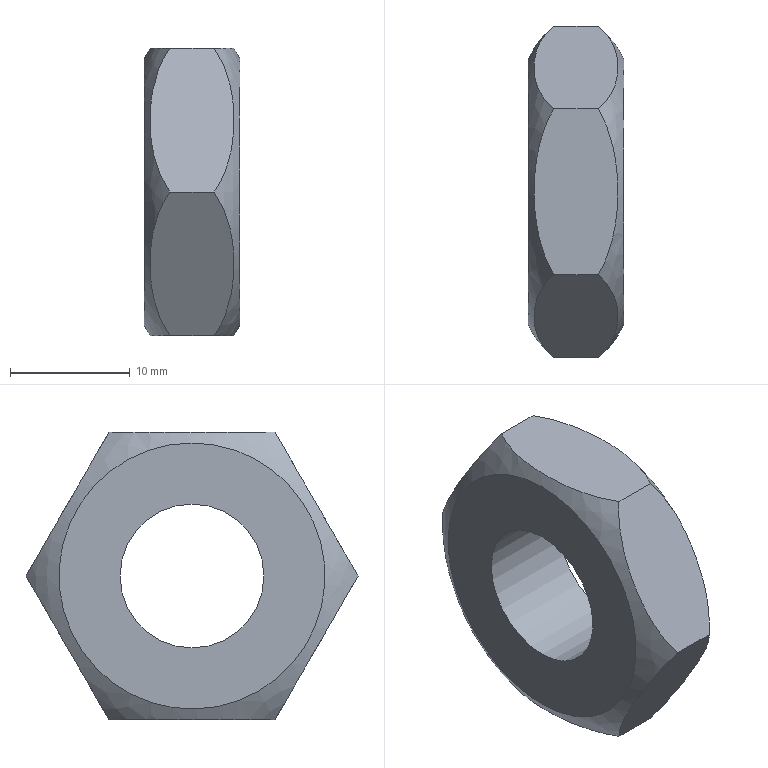Component | NX | LOCK_NUT_M12 | 1 solid | 11 faces | volume 2970 mm3 | plane 8 | spline 2 | cylinder 1 | commonest cylinder face diameters 12 x1